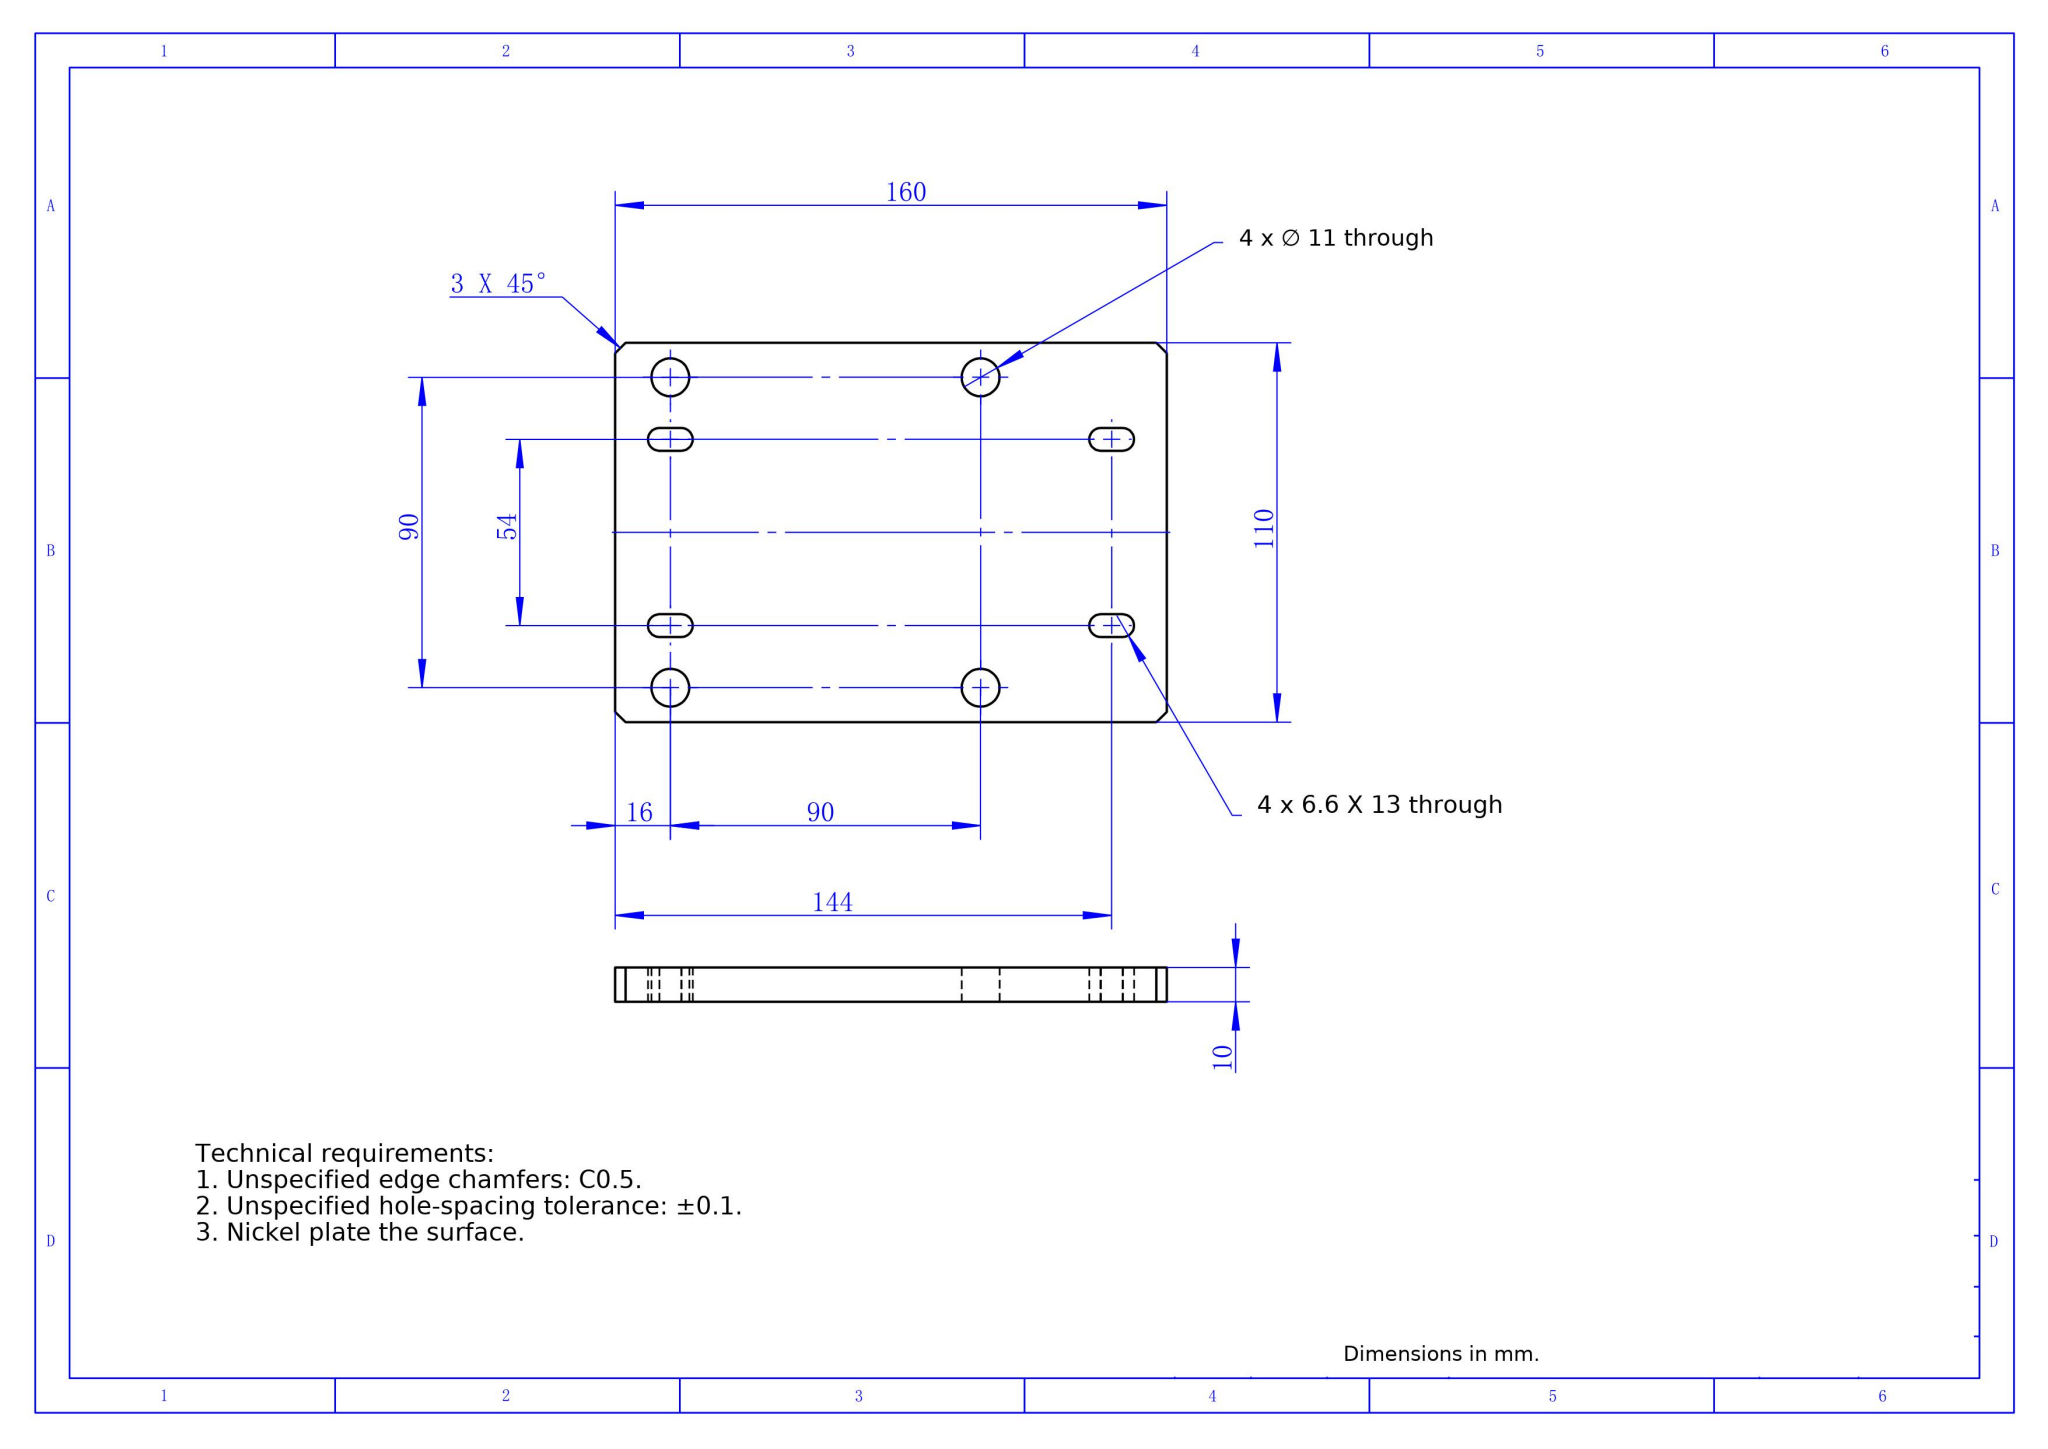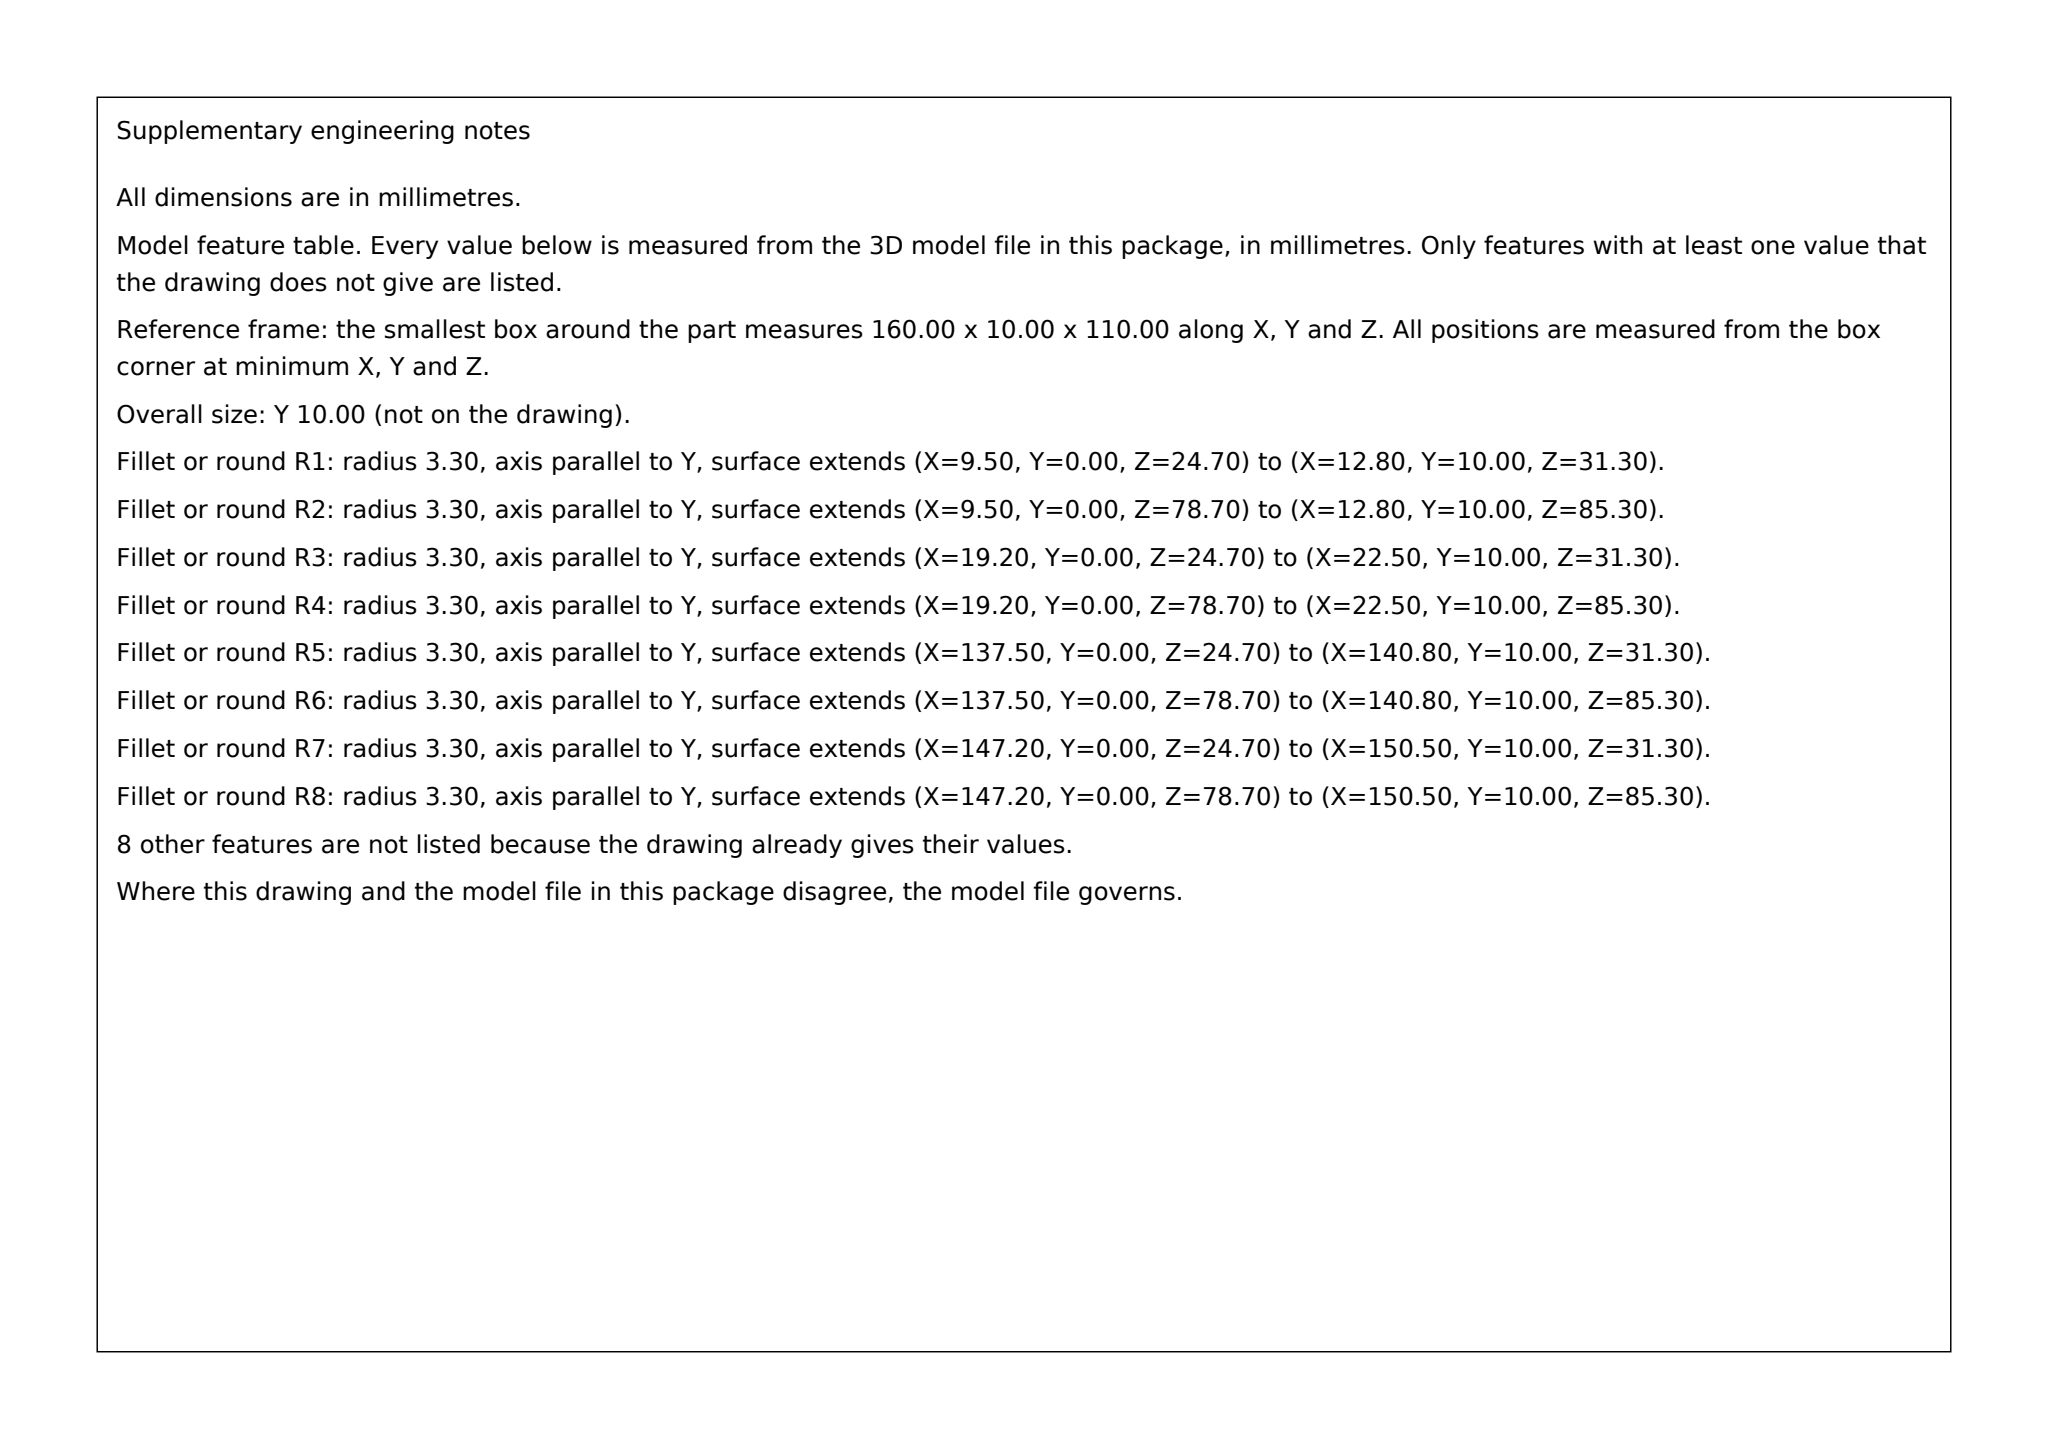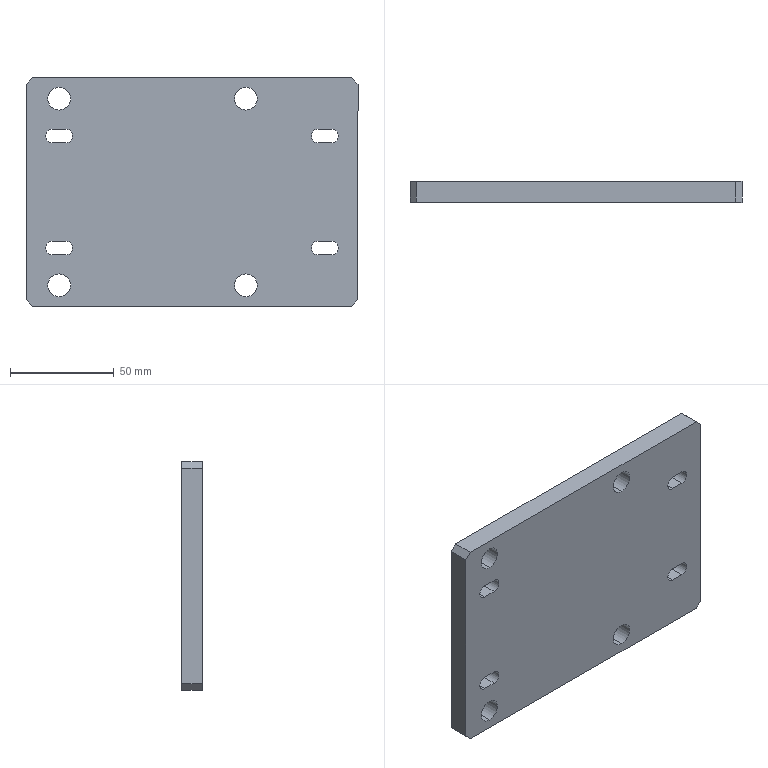Part | SolidWorks | mm | 1 solid | 34 faces | box 160 x 10 x 110 mm | volume 168961 mm3 | plane 18 | cylinder 16 | commonest cylinder face diameters 11 x8 6.6 x8